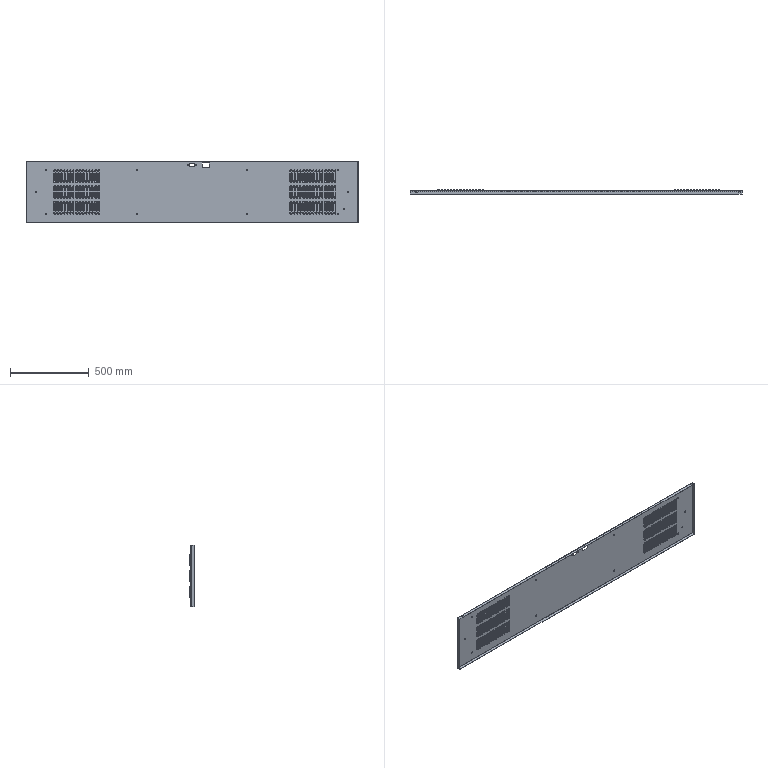Component | SolidWorks | RightRearDoorFrameAssembly-1_RightRearDoorWelding-1_RightRearDoorFrameRiveted-1_RightRearDoorFramePG50-04-101--1 | 1 solid | 2287 faces | volume 1409847 mm3 | cylinder 1142 | torus 720 | plane 425 | commonest cylinder face diameters 12.38 x270 3.02 x270 15.38 x270 0.02 x270 6 x24 9.3 x22 8.5 x4 12 x4